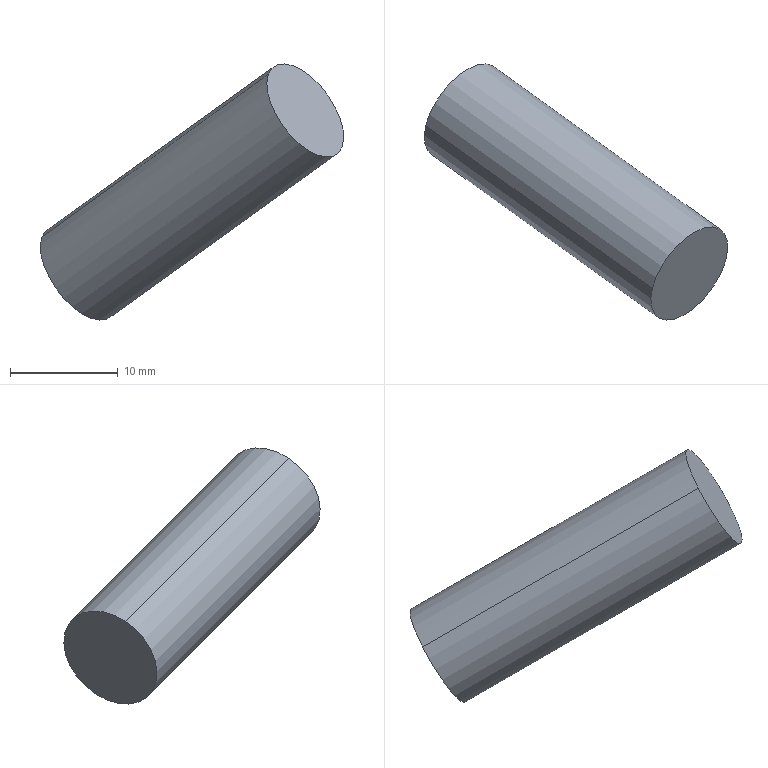Component | SolidWorks | SmallAxisAssembly-1_AdjustingWheelPivot-2 | 1 solid | 4 faces | box 28.15 x 23.78 x 23.77 mm | volume 2356 mm3 | cylinder 2 | plane 2 | commonest cylinder face diameters 10 x2
build123d program:
from build123d import *

# Parameters (mm, degrees)
SKETCH1_R           = 5
BOSS_EXTRUDE1_DEPTH = 30


with BuildPart() as part:
    # Sketch1 → Boss-Extrude1 (new body)
    with BuildSketch(Plane.XY):
        Circle(SKETCH1_R)
    extrude(amount=BOSS_EXTRUDE1_DEPTH)


solid = part.part

# Placed as in the assembly
solid = solid.moved(Location((-27.766, 778.986, 203.72), (45.029, 44.465, 44.981)))
STEP:
#1=COLOUR_RGB('',0.7922,0.8196,0.9333);
#2=FILL_AREA_STYLE_COLOUR('',#1);
#3=FILL_AREA_STYLE('',(#2));
#4=SURFACE_STYLE_FILL_AREA(#3);
#5=SURFACE_SIDE_STYLE('',(#4));
#6=SURFACE_STYLE_USAGE(.BOTH.,#5);
#7=PRESENTATION_STYLE_ASSIGNMENT((#6));
#8=CARTESIAN_POINT('',(-0.4007,30.018,8.749));
#9=VERTEX_POINT('',#8);
#10=CARTESIAN_POINT('',(-0.1309,30.127,8.484));
#11=VERTEX_POINT('',#10);
#12=CARTESIAN_POINT('',(-0.2658,30.072,8.616));
#13=DIRECTION('',(0.7005,-0.5049,0.5044));
#14=DIRECTION('',(-0.6854,-0.2788,0.6727));
#15=AXIS2_PLACEMENT_3D('',#12,#13,#14);
#16=CIRCLE('',#15,0.1969);
#17=EDGE_CURVE('',#9,#11,#16,.T.);
#18=ORIENTED_EDGE('',*,*,#17,.F.);
#19=CARTESIAN_POINT('',(-1.228,30.614,8.153));
#20=VERTEX_POINT('',#19);
#21=CARTESIAN_POINT('',(-0.4007,30.018,8.749));
#22=DIRECTION('',(-0.7005,0.5049,-0.5044));
#23=VECTOR('',#22,39.37);
#24=LINE('',#21,#23);
#25=EDGE_CURVE('',#9,#20,#24,.T.);
#26=ORIENTED_EDGE('',*,*,#25,.T.);
#27=CARTESIAN_POINT('',(-0.9582,30.724,7.888));
#28=VERTEX_POINT('',#27);
#29=CARTESIAN_POINT('',(-1.093,30.669,8.02));
#30=DIRECTION('',(0.7005,-0.5049,0.5044));
#31=DIRECTION('',(-0.6854,-0.2788,0.6727));
#32=AXIS2_PLACEMENT_3D('',#29,#30,#31);
#33=CIRCLE('',#32,0.1969);
#34=EDGE_CURVE('',#20,#28,#33,.T.);
#35=ORIENTED_EDGE('',*,*,#34,.T.);
#36=CARTESIAN_POINT('',(-0.1309,30.127,8.484));
#37=DIRECTION('',(-0.7005,0.5049,-0.5044));
#38=VECTOR('',#37,39.37);
#39=LINE('',#36,#38);
#40=EDGE_CURVE('',#11,#28,#39,.T.);
#41=ORIENTED_EDGE('',*,*,#40,.F.);
#42=EDGE_LOOP('',(#18,#26,#35,#41));
#43=FACE_OUTER_BOUND('',#42,.T.);
#44=CARTESIAN_POINT('',(-0.2658,30.072,8.616));
#45=DIRECTION('',(-0.7005,0.5049,-0.5044));
#46=DIRECTION('',(0.6854,0.2788,-0.6727));
#47=AXIS2_PLACEMENT_3D('',#44,#45,#46);
#48=CYLINDRICAL_SURFACE('',#47,0.1969);
#49=ADVANCED_FACE('',(#43),#48,.T.);
#50=ORIENTED_EDGE('',*,*,#25,.F.);
#51=CARTESIAN_POINT('',(-0.2658,30.072,8.616));
#52=DIRECTION('',(0.7005,-0.5049,0.5044));
#53=DIRECTION('',(-0.6854,-0.2788,0.6727));
#54=AXIS2_PLACEMENT_3D('',#51,#52,#53);
#55=CIRCLE('',#54,0.1969);
#56=EDGE_CURVE('',#11,#9,#55,.T.);
#57=ORIENTED_EDGE('',*,*,#56,.F.);
#58=ORIENTED_EDGE('',*,*,#40,.T.);
#59=CARTESIAN_POINT('',(-1.093,30.669,8.02));
#60=DIRECTION('',(0.7005,-0.5049,0.5044));
#61=DIRECTION('',(-0.6854,-0.2788,0.6727));
#62=AXIS2_PLACEMENT_3D('',#59,#60,#61);
#63=CIRCLE('',#62,0.1969);
#64=EDGE_CURVE('',#28,#20,#63,.T.);
#65=ORIENTED_EDGE('',*,*,#64,.T.);
#66=EDGE_LOOP('',(#50,#57,#58,#65));
#67=FACE_OUTER_BOUND('',#66,.T.);
#68=CARTESIAN_POINT('',(-0.2658,30.072,8.616));
#69=DIRECTION('',(-0.7005,0.5049,-0.5044));
#70=DIRECTION('',(0.6854,0.2788,-0.6727));
#71=AXIS2_PLACEMENT_3D('',#68,#69,#70);
#72=CYLINDRICAL_SURFACE('',#71,0.1969);
#73=ADVANCED_FACE('',(#67),#72,.T.);
#74=ORIENTED_EDGE('',*,*,#56,.T.);
#75=ORIENTED_EDGE('',*,*,#17,.T.);
#76=EDGE_LOOP('',(#74,#75));
#77=FACE_OUTER_BOUND('',#76,.T.);
#78=CARTESIAN_POINT('',(-0.2658,30.072,8.616));
#79=DIRECTION('',(0.7005,-0.5049,0.5044));
#80=DIRECTION('',(-0.6854,-0.2788,0.6727));
#81=AXIS2_PLACEMENT_3D('',#78,#79,#80);
#82=PLANE('',#81);
#83=ADVANCED_FACE('',(#77),#82,.T.);
#84=ORIENTED_EDGE('',*,*,#64,.F.);
#85=ORIENTED_EDGE('',*,*,#34,.F.);
#86=EDGE_LOOP('',(#84,#85));
#87=FACE_OUTER_BOUND('',#86,.T.);
#88=CARTESIAN_POINT('',(-1.093,30.669,8.02));
#89=DIRECTION('',(0.7005,-0.5049,0.5044));
#90=DIRECTION('',(-0.6854,-0.2788,0.6727));
#91=AXIS2_PLACEMENT_3D('',#88,#89,#90);
#92=PLANE('',#91);
#93=ADVANCED_FACE('',(#87),#92,.F.);
#94=CLOSED_SHELL('',(#49,#73,#83,#93));
#95=MANIFOLD_SOLID_BREP('',#94);
#96=STYLED_ITEM('',(#7),#95);
#97=PRESENTATION_LAYER_ASSIGNMENT('','',(#96));
#98=CARTESIAN_POINT('',(0.,0.,0.));
#99=DIRECTION('',(0.,0.,1.));
#100=DIRECTION('',(1.,0.,0.));
#101=AXIS2_PLACEMENT_3D('',#98,#99,#100);
#102=(LENGTH_UNIT()NAMED_UNIT(*)SI_UNIT($,.METRE.));
#103=LENGTH_MEASURE_WITH_UNIT(LENGTH_MEASURE(0.0254),#102);
#104=DIMENSIONAL_EXPONENTS(1.,0.,0.,0.,0.,0.,0.);
#105=(CONVERSION_BASED_UNIT('',#103)LENGTH_UNIT()NAMED_UNIT(#104));
#106=UNCERTAINTY_MEASURE_WITH_UNIT(LENGTH_MEASURE(0.00001),#105,'','');
#107=(NAMED_UNIT(*)PLANE_ANGLE_UNIT()SI_UNIT($,.RADIAN.));
#108=(NAMED_UNIT(*)SI_UNIT($,.STERADIAN.)SOLID_ANGLE_UNIT());
#109=(GEOMETRIC_REPRESENTATION_CONTEXT(3)GLOBAL_UNCERTAINTY_ASSIGNED_CONTEXT((#106))GLOBAL_UNIT_ASSIGNED_CONTEXT((#105,#107,#108))REPRESENTATION_CONTEXT('',''));
#110=ADVANCED_BREP_SHAPE_REPRESENTATION('',(#95,#101),#109);
#111=(LENGTH_UNIT()NAMED_UNIT(*)SI_UNIT($,.METRE.));
#112=LENGTH_MEASURE_WITH_UNIT(LENGTH_MEASURE(0.0254),#111);
#113=DIMENSIONAL_EXPONENTS(1.,0.,0.,0.,0.,0.,0.);
#114=(CONVERSION_BASED_UNIT('',#112)LENGTH_UNIT()NAMED_UNIT(#113));
#115=UNCERTAINTY_MEASURE_WITH_UNIT(LENGTH_MEASURE(0.00001),#114,'','');
#116=(NAMED_UNIT(*)PLANE_ANGLE_UNIT()SI_UNIT($,.RADIAN.));
#117=(NAMED_UNIT(*)SI_UNIT($,.STERADIAN.)SOLID_ANGLE_UNIT());
#118=(GEOMETRIC_REPRESENTATION_CONTEXT(3)GLOBAL_UNCERTAINTY_ASSIGNED_CONTEXT((#115))GLOBAL_UNIT_ASSIGNED_CONTEXT((#114,#116,#117))REPRESENTATION_CONTEXT('',''));
#119=MECHANICAL_DESIGN_GEOMETRIC_PRESENTATION_REPRESENTATION('',(#96),#118);